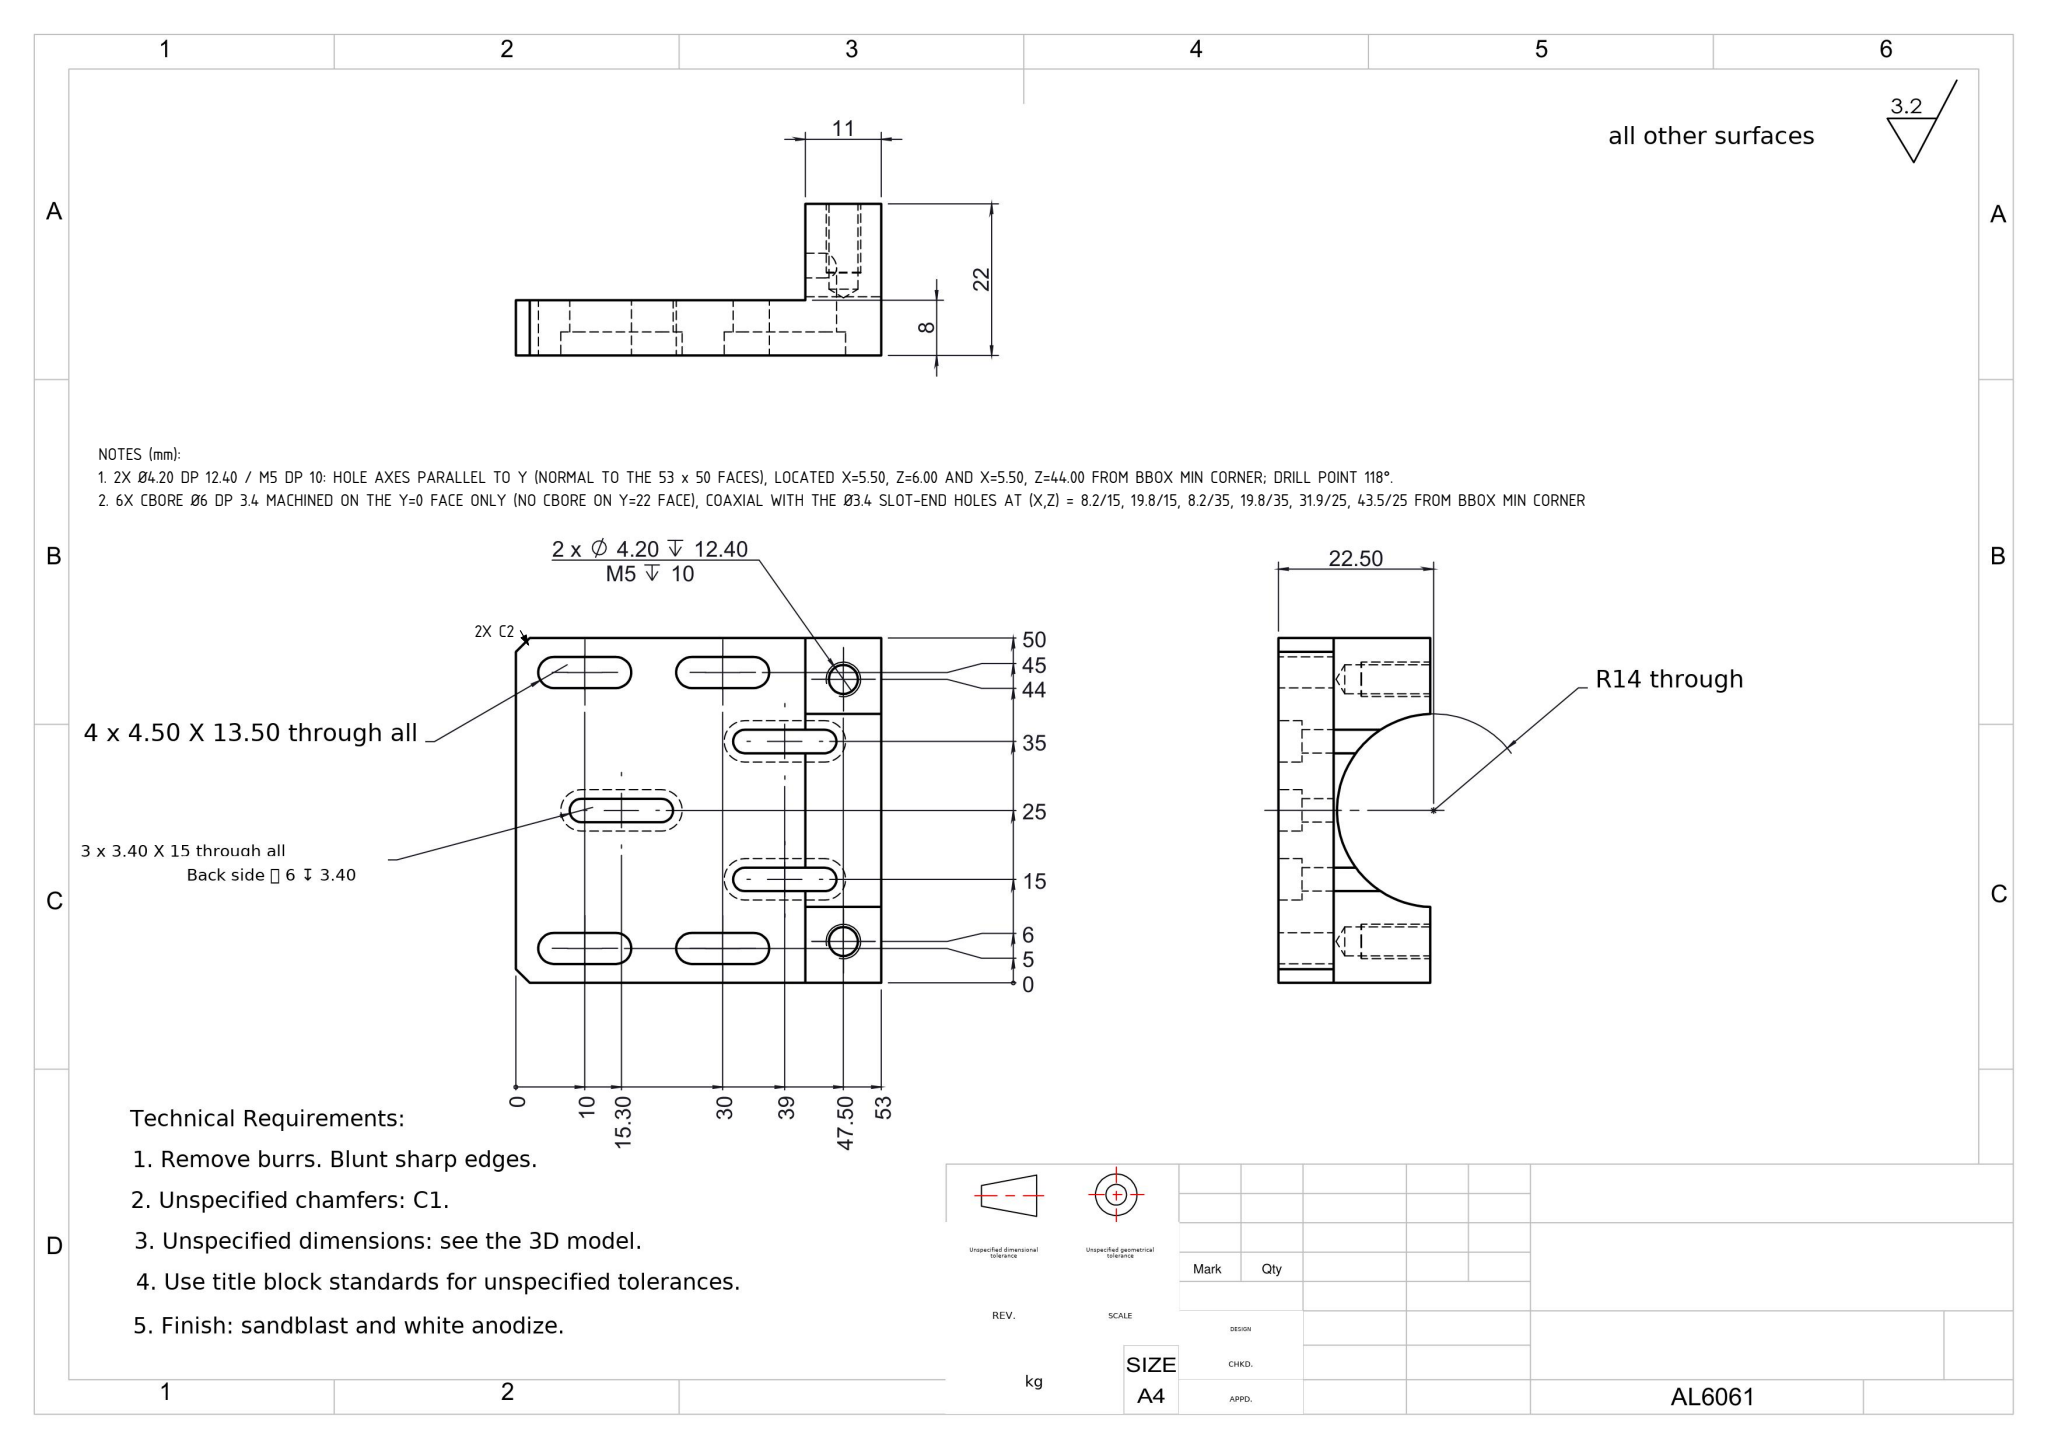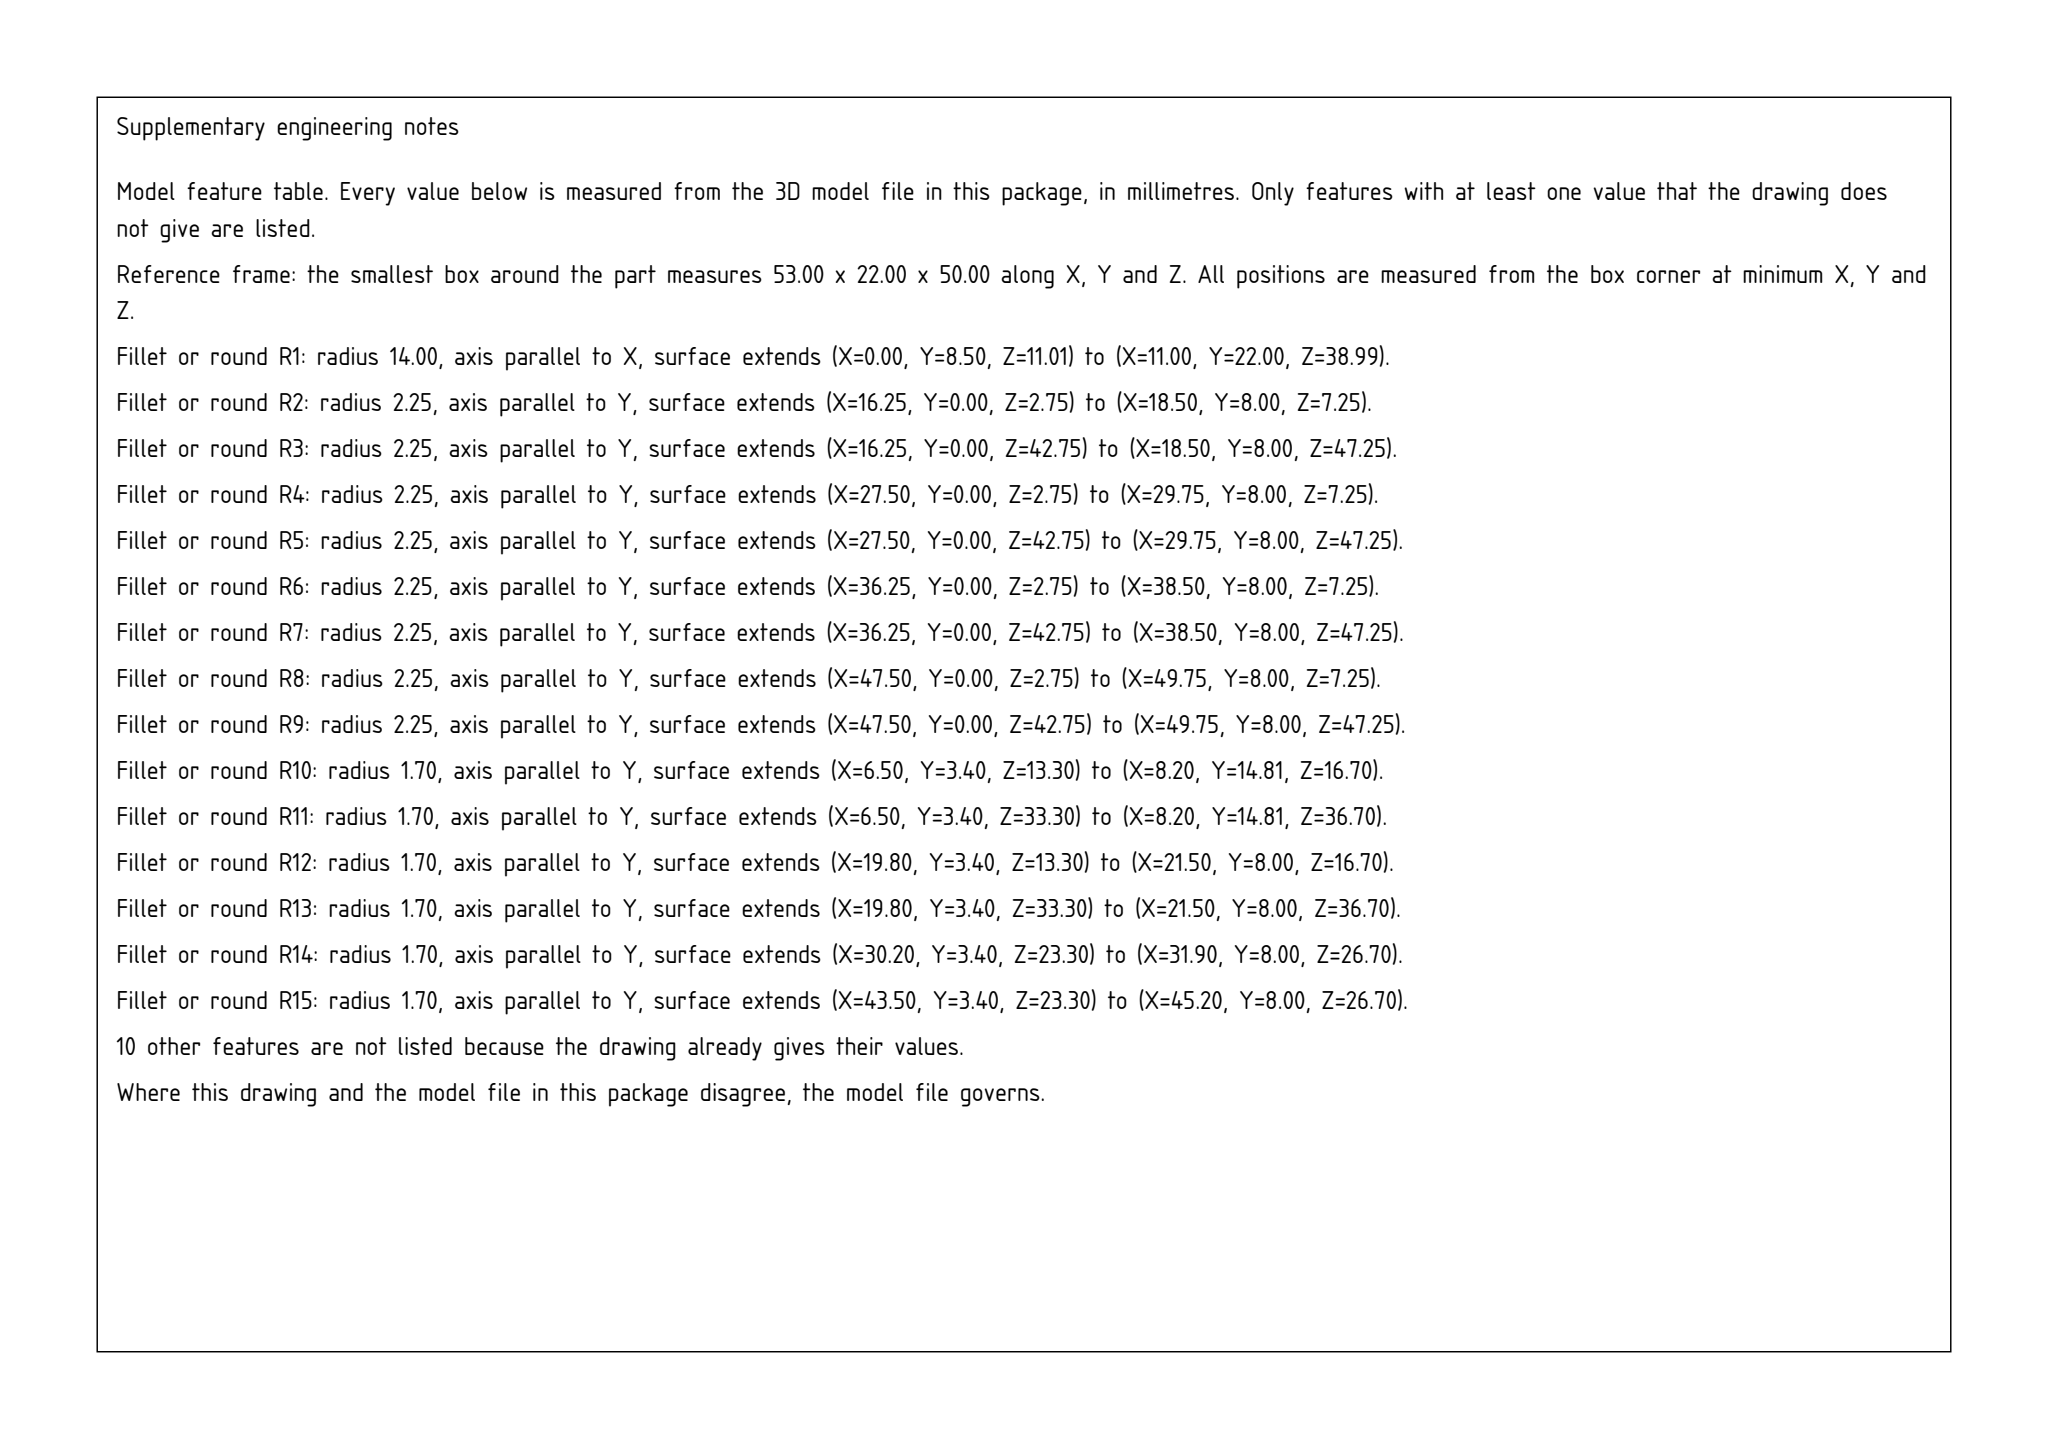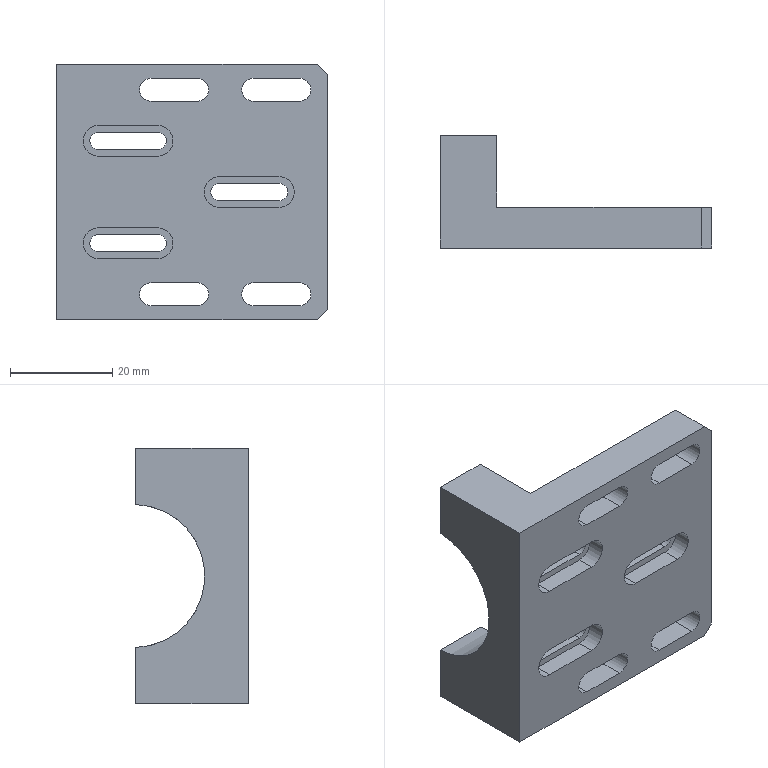Part | SolidWorks | mm | material AL6061 | 1 solid | 65 faces | box 53 x 22 x 50 mm | volume 21672 mm3 | plane 36 | cylinder 25 | cone 4 | commonest cylinder face diameters 4.5 x8 3.4 x6 6 x6 4.2 x4 28 x1
Drawing notes:
2X Ø4.20 DP 12.40 / M5 DP 10: HOLE AXES PARALLEL TO Y (NORMAL TO THE 53 x 50 FACES), LOCATED X=5.50, Z=6.00 AND X=5.50, Z=44.00 FROM BBOX MIN CORNER; DRILL POINT 118°. | from the solid: cylinders dia 4.2 axis y at (5.5,6.0) and (5.5,44.0), length 12.4; cones 118° ref dia 4.2
6X CBORE Ø6 DP 3.4 MACHINED ON THE Y=0 FACE ONLY (NO CBORE ON Y=22 FACE), COAXIAL WITH THE Ø3.4 SLOT-END HOLES AT (X,Z) = 8.2/15, 19.8/15, 8.2/35, 19.8/35, 31.9/25, 43.5/25 FROM BBOX MIN CORNER | from the solid: cylinders: six Ø6.0 bores, axis y, from y=0.0 to y=3.4 at (x,z) = (8.2,15), (19.8,15), (8.2,35), (19.8,35), (31.9,25), (43.5,25); planar faces at y=3.4 are the cbore bottoms
2X CHAMFER 2 X 45° ON THE TWO X=53 / Z=0 AND X=53 / Z=50 CORNERS OF THE 53 X 50 FACE, RUNNING FULL Y=0 TO 8 THICKNESS (CHAMFER STARTS AT X=51 AND AT Z=2 / Z=48) | from the solid: inclined_planes: two 45° faces, bbox_from [51.0,0.0,0.0] and [51.0,0.0,48.0], size [2.0,8.0,2.0]; plane x=53 extent z=[2.0,48.0]